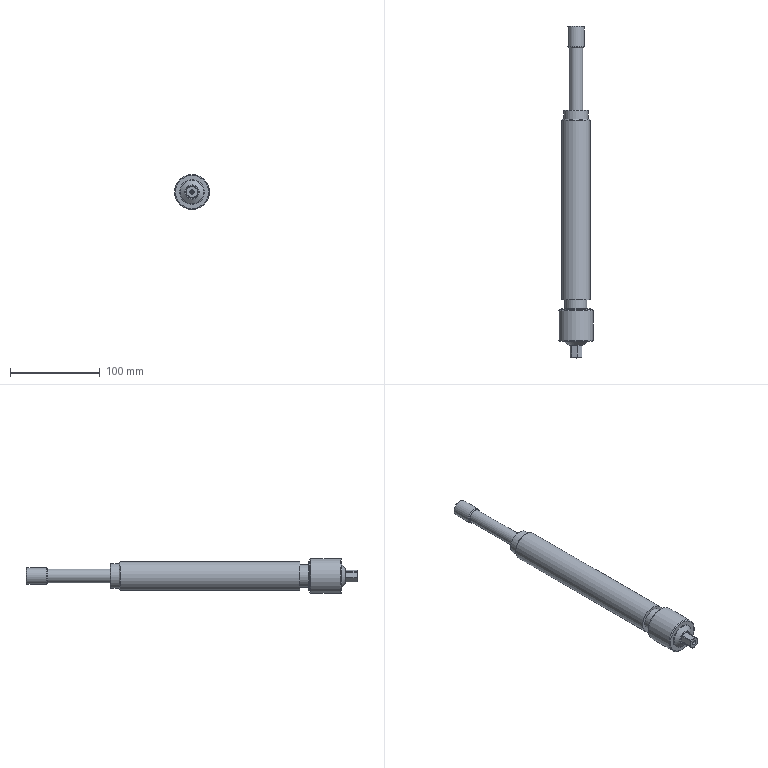Component | NX | GAN_1 | 1 solid | 45 faces | volume 236850 mm3 | plane 21 | cone 11 | cylinder 9 | torus 4 | commonest cylinder face diameters 32 x2 2.5 x2 18 x1 15 x1 27 x1 25 x1 39 x1